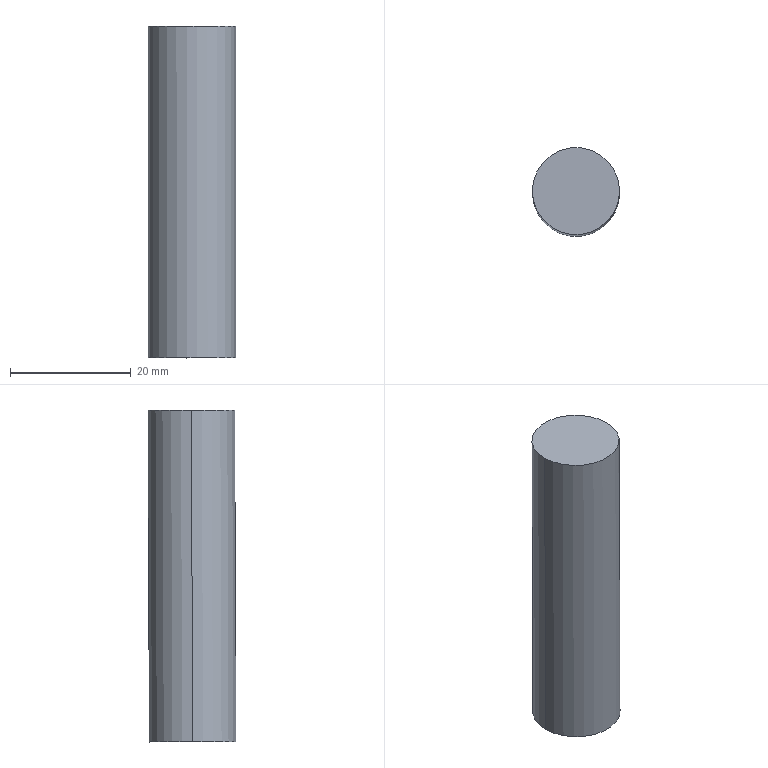Component | SolidWorks | RehabilitationChair-18-13-2 | 1 solid | 4 faces | box 14.48 x 14.67 x 55.05 mm | volume 9032 mm3 | cylinder 2 | plane 2 | commonest cylinder face diameters 14.46 x2
STEP:
#1=COLOUR_RGB('',0.7922,0.8196,0.9333);
#2=FILL_AREA_STYLE_COLOUR('',#1);
#3=FILL_AREA_STYLE('',(#2));
#4=SURFACE_STYLE_FILL_AREA(#3);
#5=SURFACE_SIDE_STYLE('',(#4));
#6=SURFACE_STYLE_USAGE(.BOTH.,#5);
#7=PRESENTATION_STYLE_ASSIGNMENT((#6));
#8=CARTESIAN_POINT('',(16.256,7.442,11.064));
#9=VERTEX_POINT('',#8);
#10=CARTESIAN_POINT('',(15.687,7.442,11.064));
#11=VERTEX_POINT('',#10);
#12=CARTESIAN_POINT('',(15.972,7.442,11.064));
#13=DIRECTION('',(0.0003323,-0.003798,-1.));
#14=DIRECTION('',(1.,0.00000716,0.0003323));
#15=AXIS2_PLACEMENT_3D('',#12,#13,#14);
#16=CIRCLE('',#15,0.2846);
#17=EDGE_CURVE('',#9,#11,#16,.T.);
#18=ORIENTED_EDGE('',*,*,#17,.F.);
#19=CARTESIAN_POINT('',(16.256,7.45,13.23));
#20=VERTEX_POINT('',#19);
#21=CARTESIAN_POINT('',(16.264,7.355,-11.688));
#22=DIRECTION('',(-0.0003323,0.003798,1.));
#23=VECTOR('',#22,39.37);
#24=LINE('',#21,#23);
#25=EDGE_CURVE('',#9,#20,#24,.T.);
#26=ORIENTED_EDGE('',*,*,#25,.T.);
#27=CARTESIAN_POINT('',(15.686,7.45,13.229));
#28=VERTEX_POINT('',#27);
#29=CARTESIAN_POINT('',(15.971,7.45,13.23));
#30=DIRECTION('',(0.0003323,-0.003798,-1.));
#31=DIRECTION('',(1.,0.00000716,0.0003323));
#32=AXIS2_PLACEMENT_3D('',#29,#30,#31);
#33=CIRCLE('',#32,0.2846);
#34=EDGE_CURVE('',#20,#28,#33,.T.);
#35=ORIENTED_EDGE('',*,*,#34,.T.);
#36=CARTESIAN_POINT('',(15.695,7.355,-11.688));
#37=DIRECTION('',(-0.0003323,0.003798,1.));
#38=VECTOR('',#37,39.37);
#39=LINE('',#36,#38);
#40=EDGE_CURVE('',#11,#28,#39,.T.);
#41=ORIENTED_EDGE('',*,*,#40,.F.);
#42=EDGE_LOOP('',(#18,#26,#35,#41));
#43=FACE_OUTER_BOUND('',#42,.T.);
#44=CARTESIAN_POINT('',(15.979,7.355,-11.688));
#45=DIRECTION('',(-0.0003323,0.003798,1.));
#46=DIRECTION('',(-1.,-0.00000716,-0.0003323));
#47=AXIS2_PLACEMENT_3D('',#44,#45,#46);
#48=CYLINDRICAL_SURFACE('',#47,0.2846);
#49=ADVANCED_FACE('',(#43),#48,.T.);
#50=CARTESIAN_POINT('',(15.972,7.442,11.064));
#51=DIRECTION('',(0.0003323,-0.003798,-1.));
#52=DIRECTION('',(1.,0.00000716,0.0003323));
#53=AXIS2_PLACEMENT_3D('',#50,#51,#52);
#54=CIRCLE('',#53,0.2846);
#55=EDGE_CURVE('',#11,#9,#54,.T.);
#56=ORIENTED_EDGE('',*,*,#55,.T.);
#57=ORIENTED_EDGE('',*,*,#17,.T.);
#58=EDGE_LOOP('',(#56,#57));
#59=FACE_OUTER_BOUND('',#58,.T.);
#60=CARTESIAN_POINT('',(23.371,23.417,11.006));
#61=DIRECTION('',(0.0003323,-0.003798,-1.));
#62=DIRECTION('',(1.,0.00000716,0.0003323));
#63=AXIS2_PLACEMENT_3D('',#60,#61,#62);
#64=PLANE('',#63);
#65=ADVANCED_FACE('',(#59),#64,.T.);
#66=ORIENTED_EDGE('',*,*,#25,.F.);
#67=ORIENTED_EDGE('',*,*,#55,.F.);
#68=ORIENTED_EDGE('',*,*,#40,.T.);
#69=CARTESIAN_POINT('',(15.971,7.45,13.23));
#70=DIRECTION('',(0.0003323,-0.003798,-1.));
#71=DIRECTION('',(1.,0.00000716,0.0003323));
#72=AXIS2_PLACEMENT_3D('',#69,#70,#71);
#73=CIRCLE('',#72,0.2846);
#74=EDGE_CURVE('',#28,#20,#73,.T.);
#75=ORIENTED_EDGE('',*,*,#74,.T.);
#76=EDGE_LOOP('',(#66,#67,#68,#75));
#77=FACE_OUTER_BOUND('',#76,.T.);
#78=CARTESIAN_POINT('',(15.979,7.355,-11.688));
#79=DIRECTION('',(-0.0003323,0.003798,1.));
#80=DIRECTION('',(-1.,-0.00000716,-0.0003323));
#81=AXIS2_PLACEMENT_3D('',#78,#79,#80);
#82=CYLINDRICAL_SURFACE('',#81,0.2846);
#83=ADVANCED_FACE('',(#77),#82,.T.);
#84=ORIENTED_EDGE('',*,*,#74,.F.);
#85=ORIENTED_EDGE('',*,*,#34,.F.);
#86=EDGE_LOOP('',(#84,#85));
#87=FACE_OUTER_BOUND('',#86,.T.);
#88=CARTESIAN_POINT('',(12.766,10.702,13.216));
#89=DIRECTION('',(0.0003323,-0.003798,-1.));
#90=DIRECTION('',(1.,0.00000716,0.0003323));
#91=AXIS2_PLACEMENT_3D('',#88,#89,#90);
#92=PLANE('',#91);
#93=ADVANCED_FACE('',(#87),#92,.F.);
#94=CLOSED_SHELL('',(#49,#65,#83,#93));
#95=MANIFOLD_SOLID_BREP('',#94);
#96=STYLED_ITEM('',(#7),#95);
#97=(LENGTH_UNIT()NAMED_UNIT(*)SI_UNIT($,.METRE.));
#98=LENGTH_MEASURE_WITH_UNIT(LENGTH_MEASURE(0.0254),#97);
#99=DIMENSIONAL_EXPONENTS(1.,0.,0.,0.,0.,0.,0.);
#100=(CONVERSION_BASED_UNIT('',#98)LENGTH_UNIT()NAMED_UNIT(#99));
#101=UNCERTAINTY_MEASURE_WITH_UNIT(LENGTH_MEASURE(0.00001),#100,'','');
#102=(NAMED_UNIT(*)PLANE_ANGLE_UNIT()SI_UNIT($,.RADIAN.));
#103=(NAMED_UNIT(*)SI_UNIT($,.STERADIAN.)SOLID_ANGLE_UNIT());
#104=(GEOMETRIC_REPRESENTATION_CONTEXT(3)GLOBAL_UNCERTAINTY_ASSIGNED_CONTEXT((#101))GLOBAL_UNIT_ASSIGNED_CONTEXT((#100,#102,#103))REPRESENTATION_CONTEXT('',''));
#105=MECHANICAL_DESIGN_GEOMETRIC_PRESENTATION_REPRESENTATION('',(#96),#104);
#106=CARTESIAN_POINT('',(0.,0.,0.));
#107=DIRECTION('',(0.,0.,1.));
#108=DIRECTION('',(1.,0.,0.));
#109=AXIS2_PLACEMENT_3D('',#106,#107,#108);
#110=(LENGTH_UNIT()NAMED_UNIT(*)SI_UNIT($,.METRE.));
#111=LENGTH_MEASURE_WITH_UNIT(LENGTH_MEASURE(0.0254),#110);
#112=DIMENSIONAL_EXPONENTS(1.,0.,0.,0.,0.,0.,0.);
#113=(CONVERSION_BASED_UNIT('',#111)LENGTH_UNIT()NAMED_UNIT(#112));
#114=UNCERTAINTY_MEASURE_WITH_UNIT(LENGTH_MEASURE(0.00001),#113,'','');
#115=(NAMED_UNIT(*)PLANE_ANGLE_UNIT()SI_UNIT($,.RADIAN.));
#116=(NAMED_UNIT(*)SI_UNIT($,.STERADIAN.)SOLID_ANGLE_UNIT());
#117=(GEOMETRIC_REPRESENTATION_CONTEXT(3)GLOBAL_UNCERTAINTY_ASSIGNED_CONTEXT((#114))GLOBAL_UNIT_ASSIGNED_CONTEXT((#113,#115,#116))REPRESENTATION_CONTEXT('',''));
#118=ADVANCED_BREP_SHAPE_REPRESENTATION('',(#95,#109),#117);
#119=PRESENTATION_LAYER_ASSIGNMENT('','',(#96));